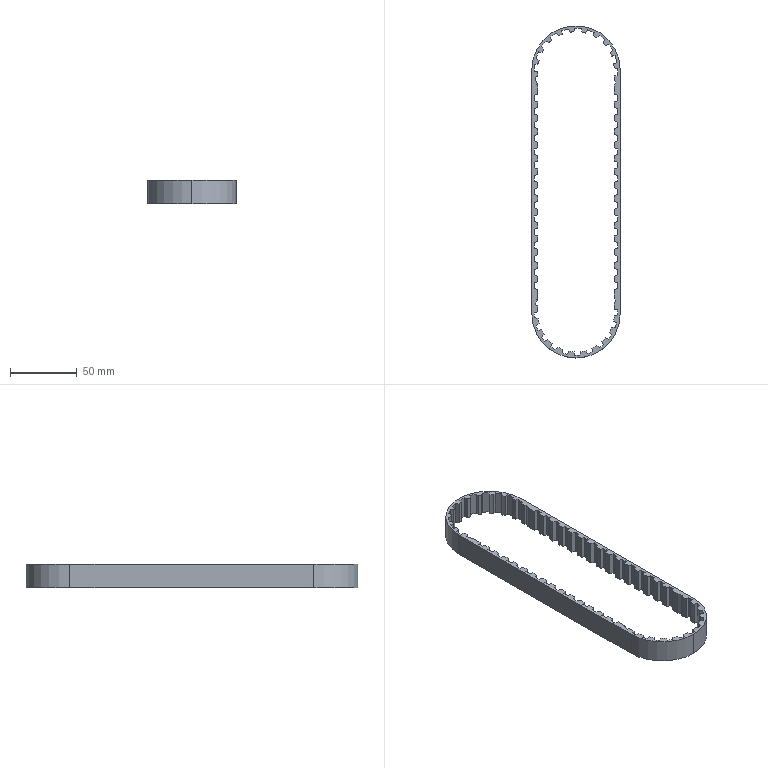Component | SolidWorks | DoubleFilmTransport-1_SynchronousBelt-1 | 1 solid | 230 faces | box 66 x 248 x 17.5 mm | volume 32341 mm3 | plane 180 | cylinder 50 | commonest cylinder face diameters 62.02 x27 57 x20 66 x3
build123d program:
from build123d import *

# Parameters (mm, degrees)
BOSS_EXTRUDE1_DEPTH = 17.5


with BuildPart() as part:
    # Sketch1 → Boss-Extrude1 (new body)
    with BuildSketch(Plane.XY.offset(8.5)):
        with BuildLine():
            Line((-91, 33), (91, 33))
            ThreePointArc((91, 33), (124, 0), (91, -33))
            Line((91, -33), (-91, -33))
            ThreePointArc((-91, -33), (-124, 0), (-91, 33))
        make_face()
        with BuildLine():
            Line((-86.531, 28.5), (-83.139, 28.5))
            Line((-83.139, 28.5), (-82.378, 29.787))
            ThreePointArc((-82.378, 29.787), (-80.558, 29.199), (-78.778, 28.5))
            Line((-78.778, 28.5), (-72.9, 28.5))
            Line((-72.9, 28.5), (-72, 31))
            Line((-72, 31), (-68, 31))
            Line((-68, 31), (-67.1, 28.5))
            Line((-67.1, 28.5), (-62.9, 28.5))
            Line((-62.9, 28.5), (-62, 31))
            Line((-62, 31), (-58, 31))
            Line((-58, 31), (-57.1, 28.5))
            Line((-57.1, 28.5), (-52.9, 28.5))
            Line((-52.9, 28.5), (-52, 31))
            Line((-52, 31), (-48, 31))
            Line((-48, 31), (-47.1, 28.5))
            Line((-47.1, 28.5), (-42.9, 28.5))
            Line((-42.9, 28.5), (-42, 31))
            Line((-42, 31), (-38, 31))
            Line((-38, 31), (-37.1, 28.5))
            Line((-37.1, 28.5), (-32.9, 28.5))
            Line((-32.9, 28.5), (-32, 31))
            Line((-32, 31), (-28, 31))
            Line((-28, 31), (-27.1, 28.5))
            Line((-27.1, 28.5), (-22.9, 28.5))
            Line((-22.9, 28.5), (-22, 31))
            Line((-22, 31), (-18, 31))
            Line((-18, 31), (-17.1, 28.5))
            Line((-17.1, 28.5), (-12.9, 28.5))
            Line((-12.9, 28.5), (-12, 31))
            Line((-12, 31), (-8, 31))
            Line((-8, 31), (-7.1, 28.5))
            Line((-7.1, 28.5), (-2.9, 28.5))
            Line((-2.9, 28.5), (-2, 31))
            Line((-2, 31), (2, 31))
            Line((2, 31), (2.9, 28.5))
            Line((2.9, 28.5), (7.1, 28.5))
            Line((7.1, 28.5), (8, 31))
            Line((8, 31), (12, 31))
            Line((12, 31), (12.9, 28.5))
            Line((12.9, 28.5), (17.1, 28.5))
            Line((17.1, 28.5), (18, 31))
            Line((18, 31), (22, 31))
            Line((22, 31), (22.9, 28.5))
            Line((22.9, 28.5), (27.1, 28.5))
            Line((27.1, 28.5), (28, 31))
            Line((28, 31), (32, 31))
            Line((32, 31), (32.9, 28.5))
            Line((32.9, 28.5), (37.1, 28.5))
            Line((37.1, 28.5), (38, 31))
            Line((38, 31), (42, 31))
            Line((42, 31), (42.9, 28.5))
            Line((42.9, 28.5), (47.1, 28.5))
            Line((47.1, 28.5), (48, 31))
            Line((48, 31), (52, 31))
            Line((52, 31), (52.9, 28.5))
            Line((52.9, 28.5), (57.1, 28.5))
            Line((57.1, 28.5), (58, 31))
            Line((58, 31), (62, 31))
            Line((62, 31), (62.9, 28.5))
            Line((62.9, 28.5), (67.1, 28.5))
            Line((67.1, 28.5), (68, 31))
            Line((68, 31), (72, 31))
            Line((72, 31), (72.9, 28.5))
            Line((72.9, 28.5), (78.778, 28.5))
            ThreePointArc((78.778, 28.5), (80.457, 29.163), (82.172, 29.727))
            Line((82.172, 29.727), (82.909, 28.5))
            Line((82.909, 28.5), (87.673, 28.5))
            Line((87.673, 28.5), (88.048, 30.869))
            ThreePointArc((88.048, 30.869), (89.917, 30.991), (91.79, 31))
            Line((91.79, 31), (92.375, 28.467))
            ThreePointArc((92.375, 28.467), (94.473, 28.288), (96.552, 27.954))
            Line((96.552, 27.954), (97.732, 30.271))
            ThreePointArc((97.732, 30.271), (99.547, 29.809), (101.331, 29.239))
            Line((101.331, 29.239), (101.104, 26.649))
            ThreePointArc((101.104, 26.649), (103.044, 25.83), (104.918, 24.87))
            Line((104.918, 24.87), (106.756, 26.709))
            ThreePointArc((106.756, 26.709), (108.34, 25.709), (109.86, 24.615))
            Line((109.86, 24.615), (108.845, 22.222))
            ThreePointArc((108.845, 22.222), (110.436, 20.844), (111.922, 19.352))
            Line((111.922, 19.352), (114.239, 20.533))
            ThreePointArc((114.239, 20.533), (115.436, 19.092), (116.544, 17.582))
            Line((116.544, 17.582), (114.838, 15.62))
            ThreePointArc((114.838, 15.62), (115.926, 13.818), (116.878, 11.94))
            Line((116.878, 11.94), (119.446, 12.346))
            ThreePointArc((119.446, 12.346), (120.14, 10.607), (120.727, 8.828))
            Line((120.727, 8.828), (118.498, 7.489))
            ThreePointArc((118.498, 7.489), (118.976, 5.439), (119.301, 3.358))
            Line((119.301, 3.358), (121.869, 2.952))
            ThreePointArc((121.869, 2.952), (121.991, 1.083), (122, -0.7899))
            Line((122, -0.7899), (119.467, -1.375))
            ThreePointArc((119.467, -1.375), (119.288, -3.473), (118.954, -5.552))
            Line((118.954, -5.552), (121.271, -6.732))
            ThreePointArc((121.271, -6.732), (120.809, -8.547), (120.239, -10.331))
            Line((120.239, -10.331), (117.649, -10.104))
            ThreePointArc((117.649, -10.104), (116.83, -12.044), (115.87, -13.918))
            Line((115.87, -13.918), (117.709, -15.756))
            ThreePointArc((117.709, -15.756), (116.709, -17.34), (115.615, -18.86))
            Line((115.615, -18.86), (113.222, -17.845))
            ThreePointArc((113.222, -17.845), (111.844, -19.436), (110.352, -20.922))
            Line((110.352, -20.922), (111.533, -23.239))
            ThreePointArc((111.533, -23.239), (110.092, -24.436), (108.582, -25.544))
            Line((108.582, -25.544), (106.62, -23.838))
            ThreePointArc((106.62, -23.838), (104.818, -24.926), (102.94, -25.878))
            Line((102.94, -25.878), (103.346, -28.446))
            ThreePointArc((103.346, -28.446), (101.607, -29.14), (99.828, -29.727))
            Line((99.828, -29.727), (98.489, -27.498))
            ThreePointArc((98.489, -27.498), (96.439, -27.976), (94.358, -28.301))
            Line((94.358, -28.301), (93.952, -30.869))
            ThreePointArc((93.952, -30.869), (92.083, -30.991), (90.21, -31))
            Line((90.21, -31), (89.633, -28.5))
            Line((89.633, -28.5), (85.17, -28.5))
            Line((85.17, -28.5), (84.268, -30.271))
            ThreePointArc((84.268, -30.271), (82.453, -29.809), (80.669, -29.239))
            Line((80.669, -29.239), (80.734, -28.5))
            Line((80.734, -28.5), (72.9, -28.5))
            Line((72.9, -28.5), (72, -31))
            Line((72, -31), (68, -31))
            Line((68, -31), (67.1, -28.5))
            Line((67.1, -28.5), (62.9, -28.5))
            Line((62.9, -28.5), (62, -31))
            Line((62, -31), (58, -31))
            Line((58, -31), (57.1, -28.5))
            Line((57.1, -28.5), (52.9, -28.5))
            Line((52.9, -28.5), (52, -31))
            Line((52, -31), (48, -31))
            Line((48, -31), (47.1, -28.5))
            Line((47.1, -28.5), (42.9, -28.5))
            Line((42.9, -28.5), (42, -31))
            Line((42, -31), (38, -31))
            Line((38, -31), (37.1, -28.5))
            Line((37.1, -28.5), (32.9, -28.5))
            Line((32.9, -28.5), (32, -31))
            Line((32, -31), (28, -31))
            Line((28, -31), (27.1, -28.5))
            Line((27.1, -28.5), (22.9, -28.5))
            Line((22.9, -28.5), (22, -31))
            Line((22, -31), (18, -31))
            Line((18, -31), (17.1, -28.5))
            Line((17.1, -28.5), (12.9, -28.5))
            Line((12.9, -28.5), (12, -31))
            Line((12, -31), (8, -31))
            Line((8, -31), (7.1, -28.5))
            Line((7.1, -28.5), (2.9, -28.5))
            Line((2.9, -28.5), (2, -31))
            Line((2, -31), (-2, -31))
            Line((-2, -31), (-2.9, -28.5))
            Line((-2.9, -28.5), (-7.1, -28.5))
            Line((-7.1, -28.5), (-8, -31))
            Line((-8, -31), (-12, -31))
            Line((-12, -31), (-12.9, -28.5))
            Line((-12.9, -28.5), (-17.1, -28.5))
            Line((-17.1, -28.5), (-18, -31))
            Line((-18, -31), (-22, -31))
            Line((-22, -31), (-22.9, -28.5))
            Line((-22.9, -28.5), (-27.1, -28.5))
            Line((-27.1, -28.5), (-28, -31))
            Line((-28, -31), (-32, -31))
            Line((-32, -31), (-32.9, -28.5))
            Line((-32.9, -28.5), (-37.1, -28.5))
            Line((-37.1, -28.5), (-38, -31))
            Line((-38, -31), (-42, -31))
            Line((-42, -31), (-42.9, -28.5))
            Line((-42.9, -28.5), (-47.1, -28.5))
            Line((-47.1, -28.5), (-48, -31))
            Line((-48, -31), (-52, -31))
            Line((-52, -31), (-52.9, -28.5))
            Line((-52.9, -28.5), (-57.1, -28.5))
            Line((-57.1, -28.5), (-58, -31))
            Line((-58, -31), (-62, -31))
            Line((-62, -31), (-62.9, -28.5))
            Line((-62.9, -28.5), (-67.1, -28.5))
            Line((-67.1, -28.5), (-68, -31))
            Line((-68, -31), (-72, -31))
            Line((-72, -31), (-72.9, -28.5))
            Line((-72.9, -28.5), (-80.53, -28.5))
            Line((-80.53, -28.5), (-80.467, -29.166))
            ThreePointArc((-80.467, -29.166), (-82.959, -29.949), (-85.509, -30.52))
            Line((-85.509, -30.52), (-86.436, -28.5))
            Line((-86.436, -28.5), (-89.438, -28.5))
            Line((-89.438, -28.5), (-89.995, -30.994))
            ThreePointArc((-89.995, -30.994), (-92.608, -30.968), (-95.209, -30.723))
            Line((-95.209, -30.723), (-95.51, -28.141))
            ThreePointArc((-95.51, -28.141), (-96.912, -27.88), (-98.298, -27.55))
            Line((-98.298, -27.55), (-99.622, -29.787))
            ThreePointArc((-99.622, -29.787), (-102.099, -28.956), (-104.497, -27.919))
            Line((-104.497, -27.919), (-103.986, -25.37))
            ThreePointArc((-103.986, -25.37), (-105.238, -24.689), (-106.455, -23.946))
            Line((-106.455, -23.946), (-108.405, -25.665))
            ThreePointArc((-108.405, -25.665), (-110.503, -24.109), (-112.464, -22.382))
            Line((-112.464, -22.382), (-111.19, -20.115))
            ThreePointArc((-111.19, -20.115), (-112.17, -19.081), (-113.098, -17.998))
            Line((-113.098, -17.998), (-115.484, -19.031))
            ThreePointArc((-115.484, -19.031), (-116.999, -16.902), (-118.329, -14.653))
            Line((-118.329, -14.653), (-116.418, -12.892))
            ThreePointArc((-116.418, -12.892), (-117.03, -11.605), (-117.578, -10.289))
            Line((-117.578, -10.289), (-120.166, -10.533))
            ThreePointArc((-120.166, -10.533), (-120.949, -8.041), (-121.52, -5.491))
            Line((-121.52, -5.491), (-119.157, -4.406))
            ThreePointArc((-119.157, -4.406), (-119.342, -2.993), (-119.457, -1.572))
            Line((-119.457, -1.572), (-121.994, -1.005))
            ThreePointArc((-121.994, -1.005), (-121.968, 1.608), (-121.723, 4.209))
            Line((-121.723, 4.209), (-119.141, 4.51))
            ThreePointArc((-119.141, 4.51), (-118.88, 5.912), (-118.55, 7.298))
            Line((-118.55, 7.298), (-120.787, 8.622))
            ThreePointArc((-120.787, 8.622), (-119.956, 11.099), (-118.919, 13.497))
            Line((-118.919, 13.497), (-116.37, 12.986))
            ThreePointArc((-116.37, 12.986), (-115.689, 14.238), (-114.946, 15.455))
            Line((-114.946, 15.455), (-116.665, 17.405))
            ThreePointArc((-116.665, 17.405), (-115.109, 19.503), (-113.382, 21.464))
            Line((-113.382, 21.464), (-111.115, 20.19))
            ThreePointArc((-111.115, 20.19), (-110.081, 21.17), (-108.998, 22.098))
            Line((-108.998, 22.098), (-110.031, 24.484))
            ThreePointArc((-110.031, 24.484), (-107.902, 25.999), (-105.653, 27.329))
            Line((-105.653, 27.329), (-103.892, 25.418))
            ThreePointArc((-103.892, 25.418), (-102.605, 26.03), (-101.289, 26.578))
            Line((-101.289, 26.578), (-101.533, 29.166))
            ThreePointArc((-101.533, 29.166), (-99.041, 29.949), (-96.491, 30.52))
            Line((-96.491, 30.52), (-95.406, 28.157))
            ThreePointArc((-95.406, 28.157), (-93.993, 28.342), (-92.572, 28.457))
            Line((-92.572, 28.457), (-92.005, 30.994))
            ThreePointArc((-92.005, 30.994), (-89.392, 30.968), (-86.791, 30.723))
            Line((-86.791, 30.723), (-86.531, 28.5))
        make_face(mode=Mode.SUBTRACT)
    extrude(amount=-BOSS_EXTRUDE1_DEPTH)


solid = part.part

# Placed as in the assembly
solid = solid.moved(Location((-384.677, 174.373, 116), (0, 0, -90)))